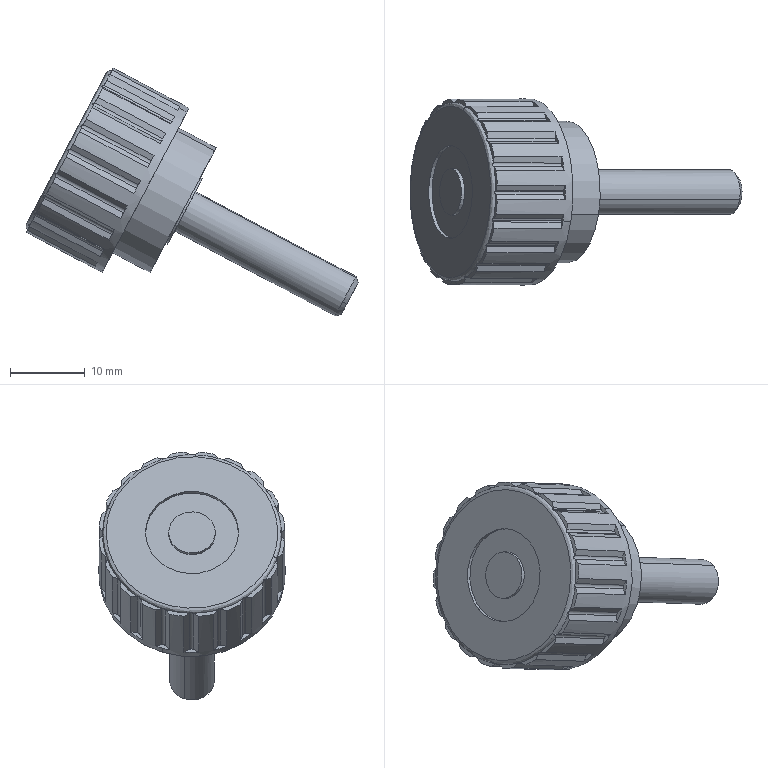Component | SolidWorks | NBM6_25_25_B_NBM6-25-25-B-2 | 1 solid | 126 faces | volume 8038 mm3 | plane 87 | cylinder 35 | spline 2 | cone 2 | commonest cylinder face diameters 1 x23 12.5 x2 25 x2 6.25 x2 19 x2 10 x2 6 x2